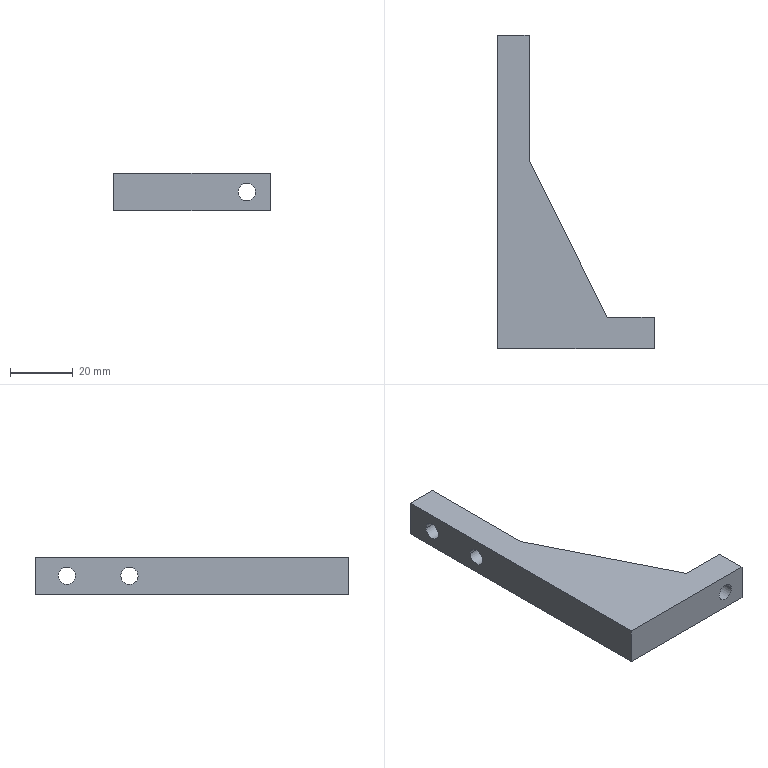CAM job | Mastercam | mm | 13 operations | part box 50 x 100 x 12
1. Facing | 24 - 100 平铣刀
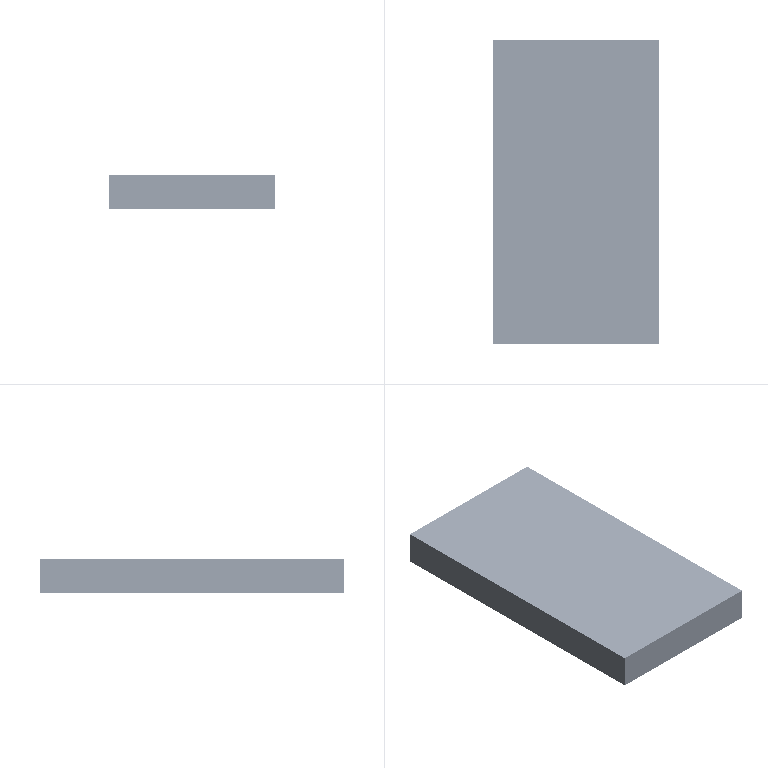2. 2D High Speed (2D Dynamic Mill) | 12 - 12 平铣刀
3. Contour (2D) | 12 - 12 平铣刀
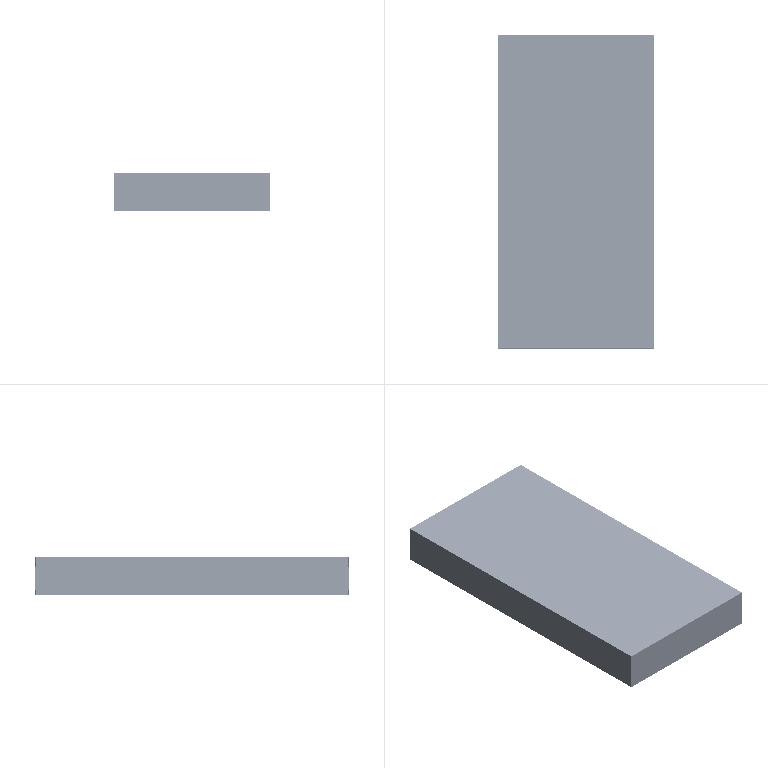4. Contour (2D chamfer) | 7 - 4 倒角刀
5. Facing | 24 - 100 平铣刀
6. Contour (2D chamfer) | 7 - 4 倒角刀
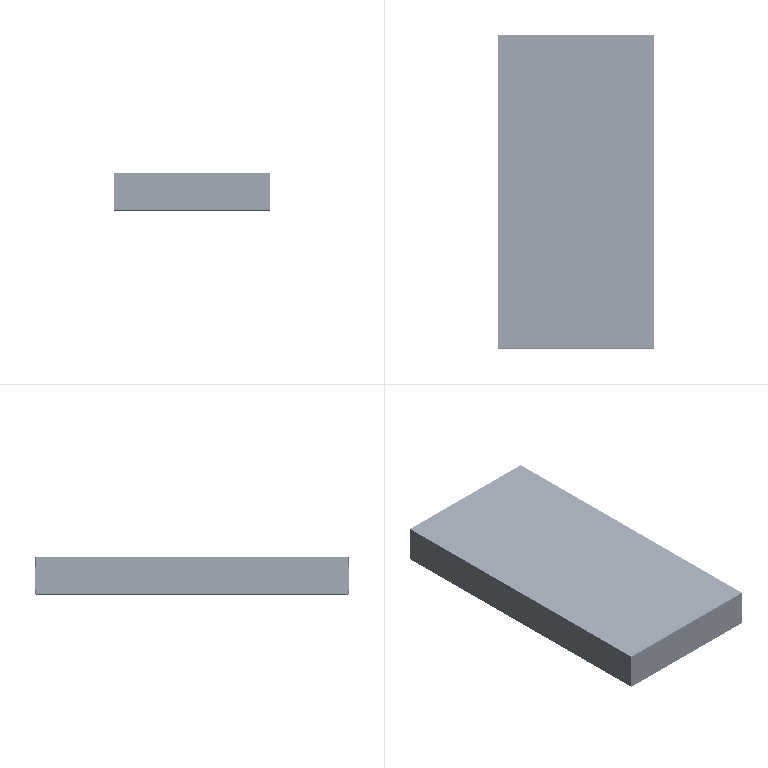7. Drill/Counterbore | 7 - 4 倒角刀
8. 3D High Speed (Area roughing) | 12 - 12 平铣刀
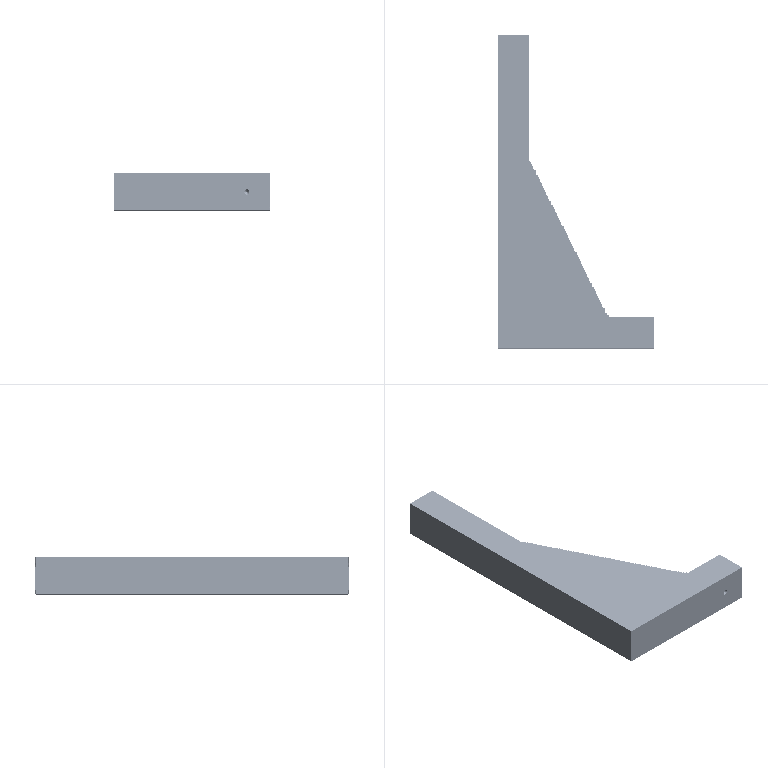9. Contour (2D) | 12 - 12 平铣刀
10. Contour (2D) | 12 - 12 平铣刀
11. Surface Finish Flowline | 12 - 12 平铣刀
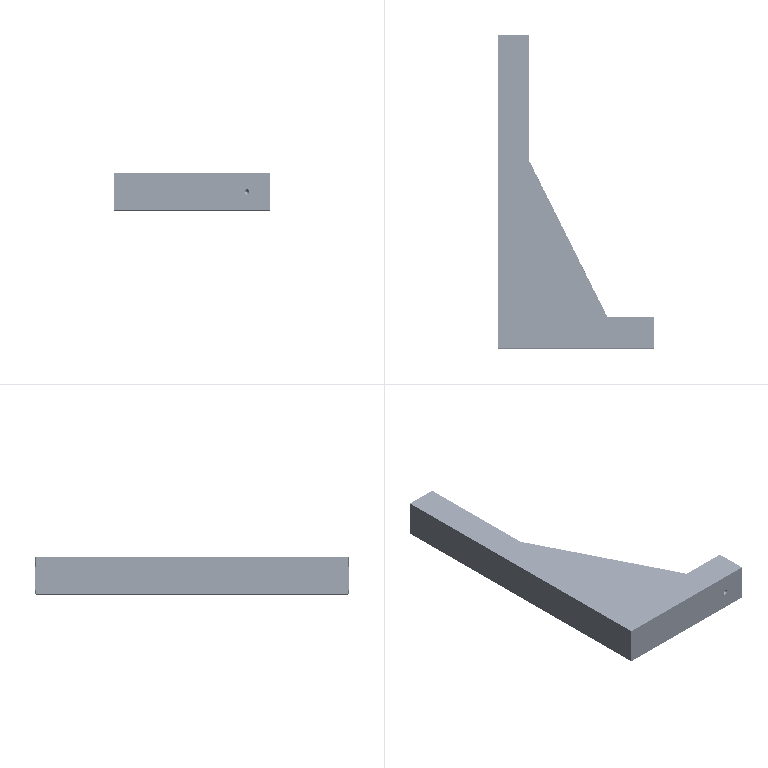12. Drill/Counterbore | 7 - 4 倒角刀
13. Contour (2D chamfer) | 7 - 4 倒角刀